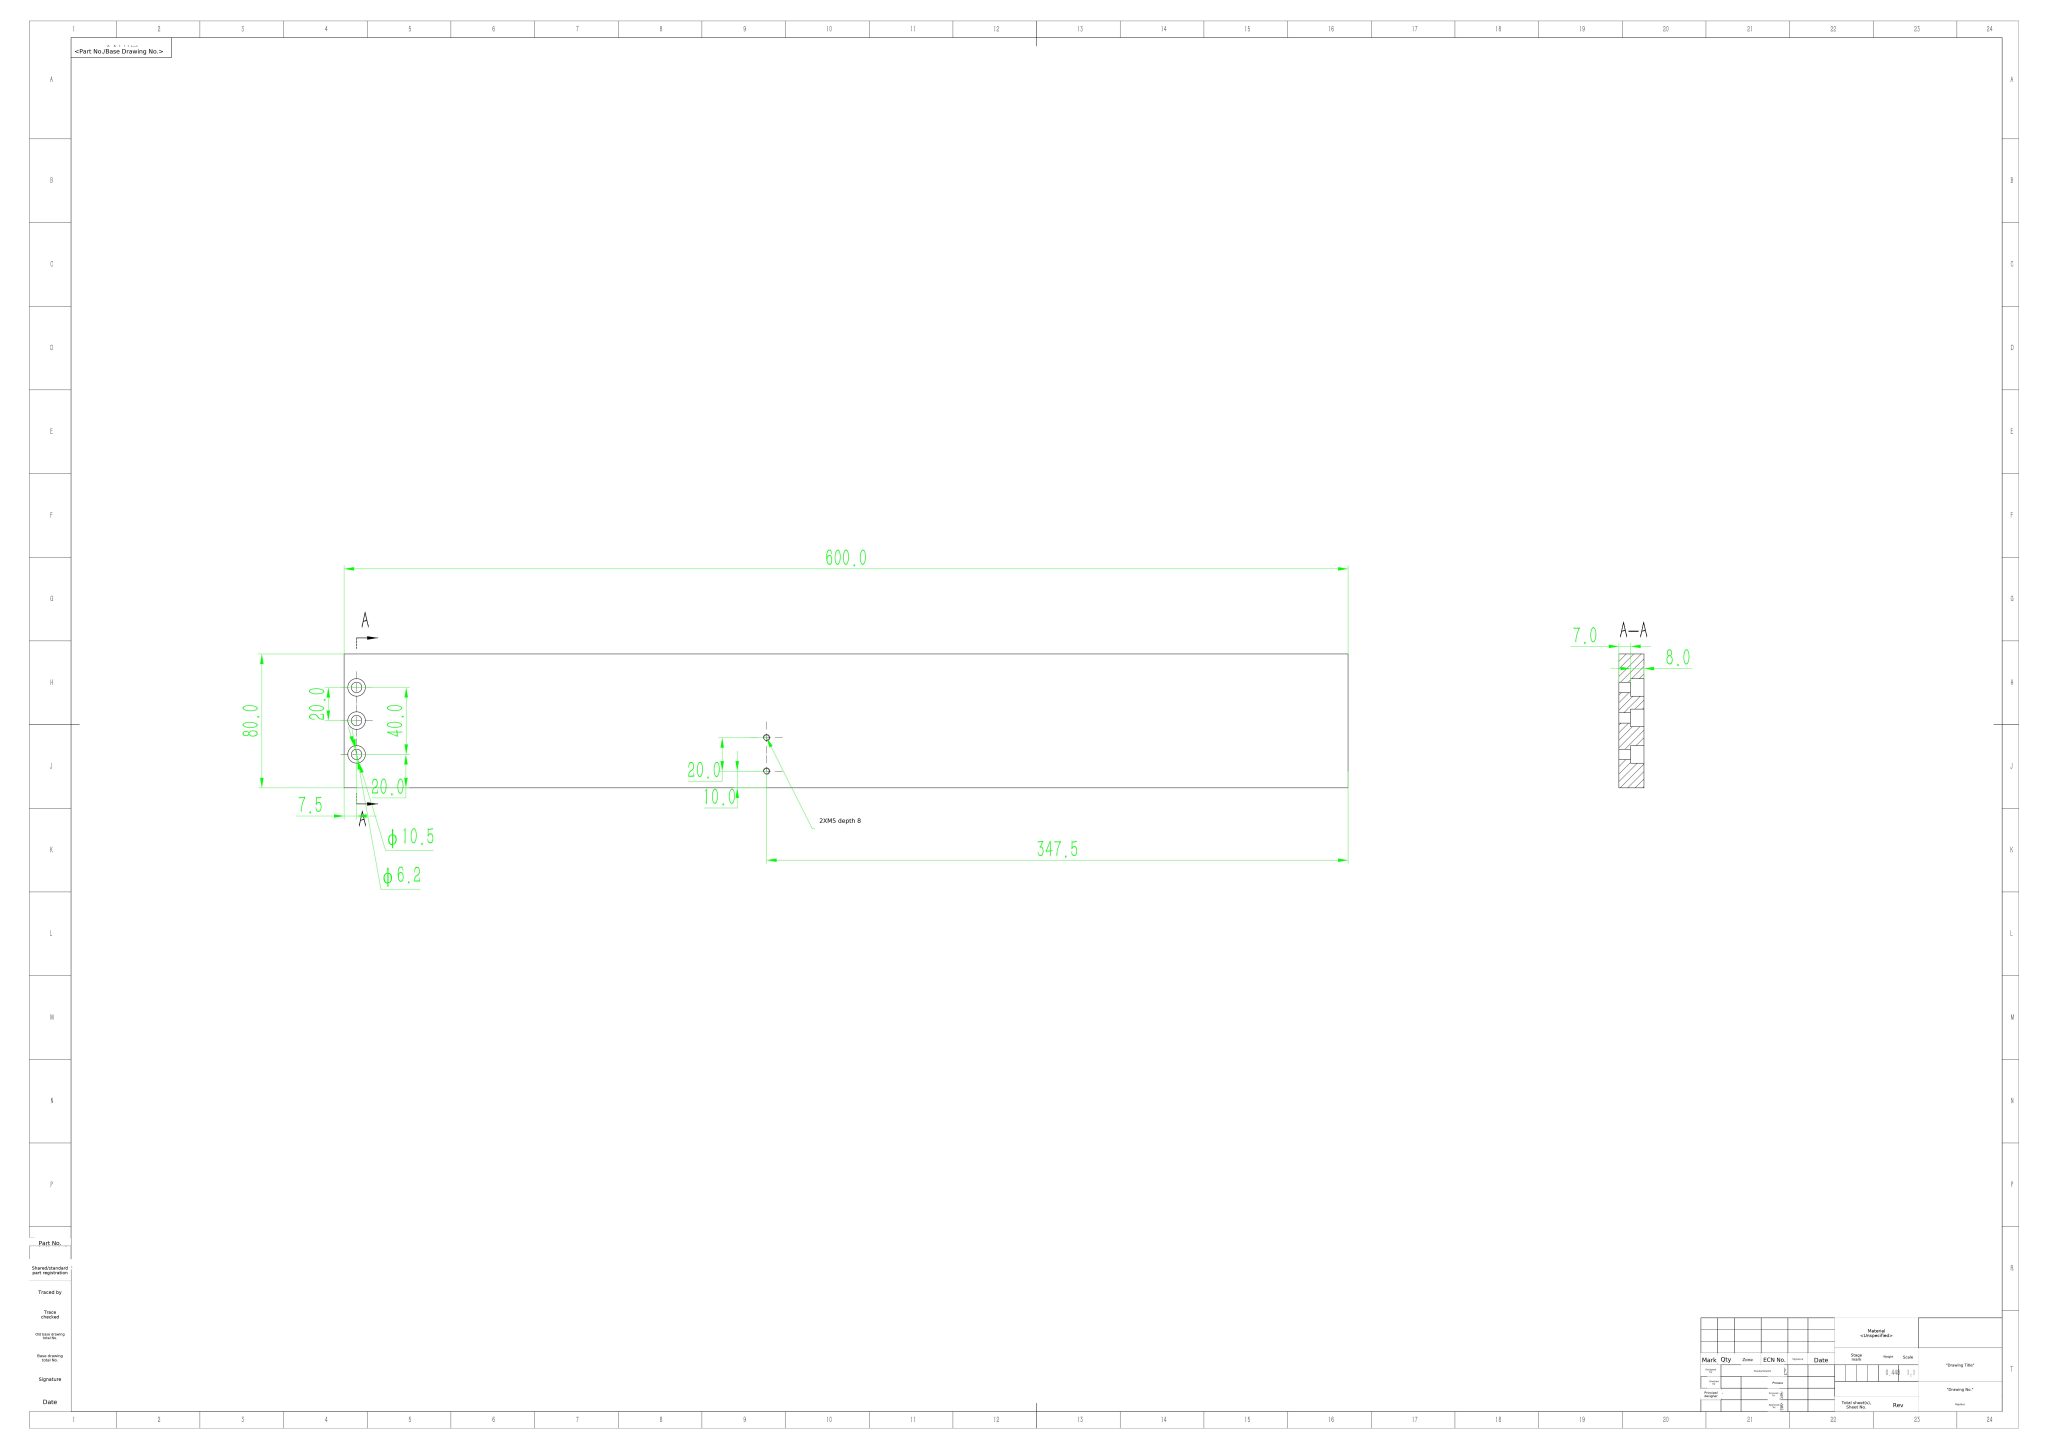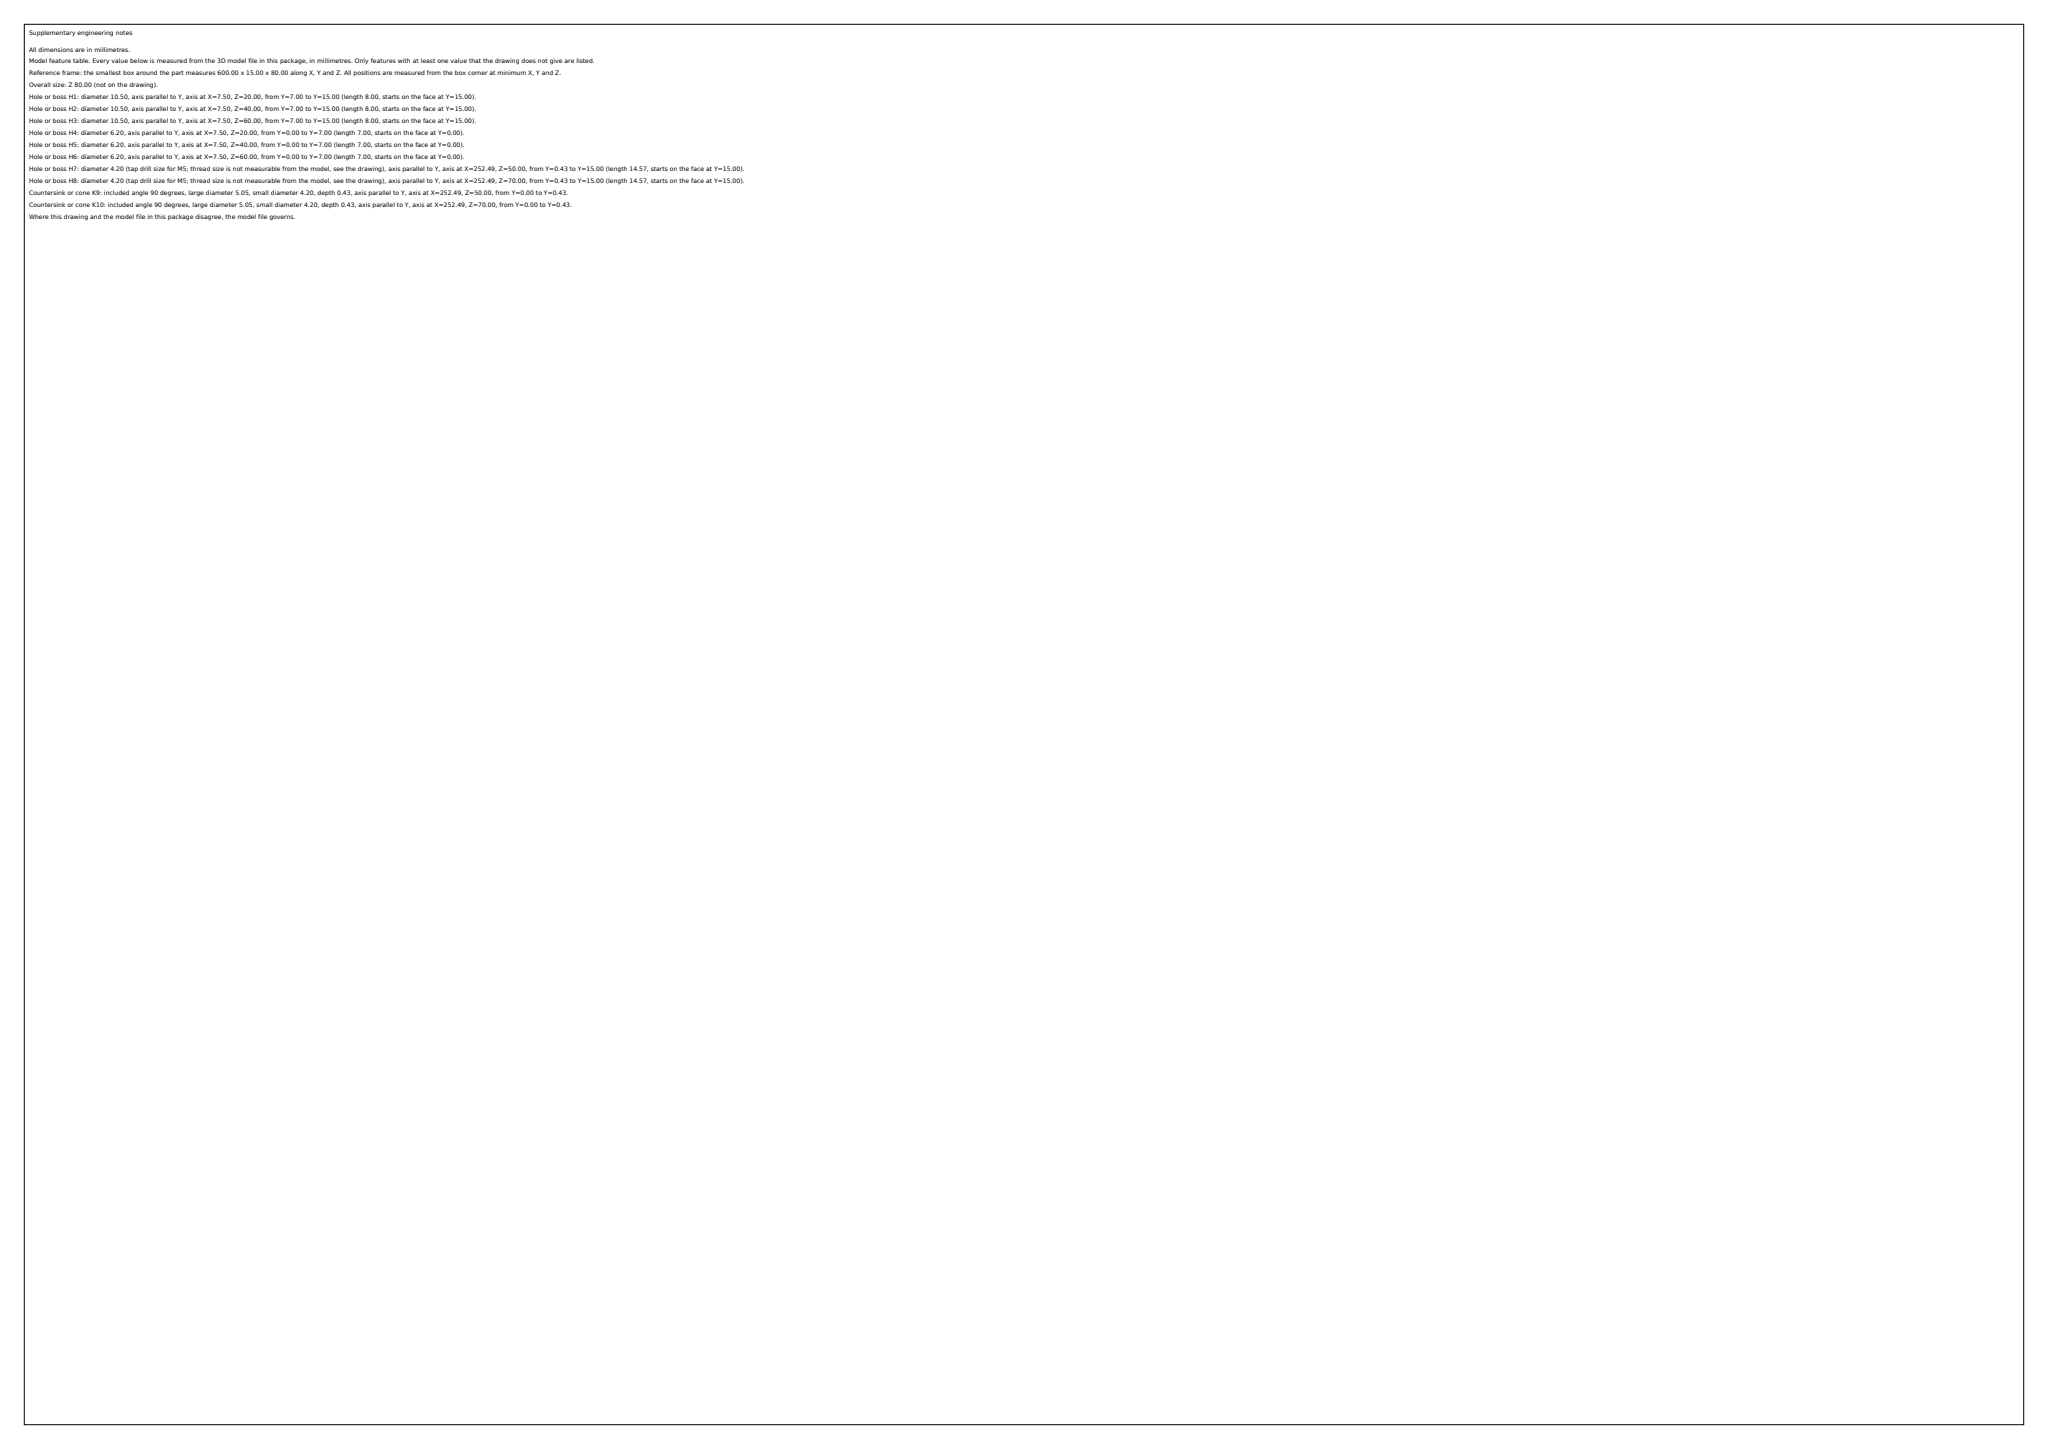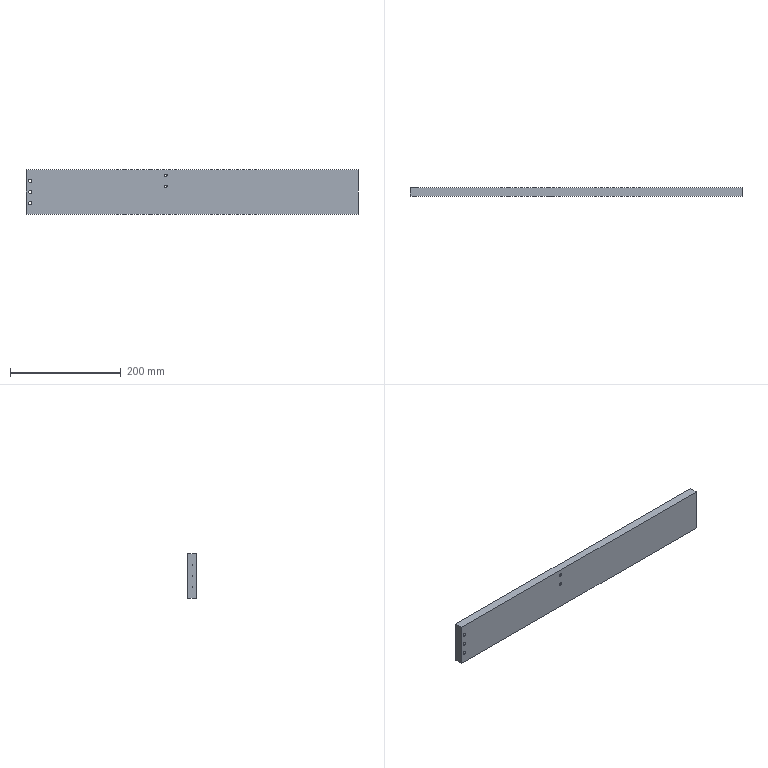Part | SolidWorks | mm | 1 solid | 29 faces | box 600 x 15 x 80 mm | volume 716870 mm3 | cylinder 16 | plane 9 | cone 4 | commonest cylinder face diameters 6.2 x6 10.5 x6 4.2 x4
build123d program:
from build123d import *

# Parameters (mm, degrees)
SKETCH1_W                   = 600
SKETCH1_H                   = 80
BOSS_EXTRUDE1_DEPTH         = 15
SKETCH2_R                   = 5.25
CUT_EXTRUDE1_DEPTH          = 8
SKETCH3_R                   = 3.1
CUT_EXTRUDE2_DEPTH          = 303.761
M5_TAPPED_HOLE1_D           = 4.2
M5_TAPPED_HOLE1_CSINK_D     = 5.05
M5_TAPPED_HOLE1_CSINK_ANGLE = 90


with BuildPart() as part:
    # Sketch1 → Boss-Extrude1 (new body)
    with BuildSketch(Plane(origin=(0, 0, 0), x_dir=(1, 0, 0), z_dir=(0, 1, 0))):
        Rectangle(SKETCH1_W, SKETCH1_H)
    extrude(amount=BOSS_EXTRUDE1_DEPTH)

    # Sketch2 → Cut-Extrude1 (cut)
    with BuildSketch(Plane(origin=(0, 15, 0), x_dir=(1, 0, 0), z_dir=(0, 1, 0))):
        with Locations(Location((-292.5, 20, 0), (0, 0, 270))):
            Circle(SKETCH2_R)
        with Locations(Location((-292.5, -20, 0), (0, 0, 270))):
            Circle(SKETCH2_R)
        with Locations(Location((-292.5, 0, 0), (0, 0, 270))):
            Circle(SKETCH2_R)
    extrude(amount=-CUT_EXTRUDE1_DEPTH, mode=Mode.SUBTRACT)

    # Sketch3 → Cut-Extrude2 (cut, through all)
    with BuildSketch(Plane(origin=(0, 7, 0), x_dir=(1, 0, 0), z_dir=(0, 1, 0))):
        with Locations(Location((-292.5, 20, 0), (0, 0, 270))):
            Circle(SKETCH3_R)
        with Locations(Location((-292.5, -20, 0), (0, 0, 270))):
            Circle(SKETCH3_R)
        with Locations(Location((-292.5, 0, 0), (0, 0, 270))):
            Circle(SKETCH3_R)
    extrude(amount=-CUT_EXTRUDE2_DEPTH, mode=Mode.SUBTRACT)

    # M5 Tapped Hole1 (through all)
    with Locations(Plane(origin=(0, 0, 0), x_dir=(-1, 0, 0), z_dir=(0, -1, 0))):
        with Locations((47.513, -30), (47.513, -10)):
            CounterSinkHole(M5_TAPPED_HOLE1_D / 2, M5_TAPPED_HOLE1_CSINK_D / 2, counter_sink_angle=M5_TAPPED_HOLE1_CSINK_ANGLE)


solid = part.part
STEP:
#1=CARTESIAN_POINT('',(-47.513,0.425,32.1));
#2=VERTEX_POINT('',#1);
#3=CARTESIAN_POINT('',(-47.513,0.425,27.9));
#4=VERTEX_POINT('',#3);
#5=CARTESIAN_POINT('',(-47.513,0.425,30.));
#6=DIRECTION('',(0.,-1.,0.));
#7=DIRECTION('',(0.,0.,-1.));
#8=AXIS2_PLACEMENT_3D('',#5,#6,#7);
#9=CIRCLE('',#8,2.1);
#10=EDGE_CURVE('',#2,#4,#9,.T.);
#11=ORIENTED_EDGE('',*,*,#10,.F.);
#12=CARTESIAN_POINT('',(-47.513,-0.,32.525));
#13=VERTEX_POINT('',#12);
#14=CARTESIAN_POINT('',(-47.513,-0.,32.525));
#15=DIRECTION('',(0.,-0.7071,0.7071));
#16=VECTOR('',#15,1000.);
#17=LINE('',#14,#16);
#18=EDGE_CURVE('',#2,#13,#17,.T.);
#19=ORIENTED_EDGE('',*,*,#18,.T.);
#20=CARTESIAN_POINT('',(-47.513,-0.,27.475));
#21=VERTEX_POINT('',#20);
#22=CARTESIAN_POINT('',(-47.513,-0.,30.));
#23=DIRECTION('',(0.,-1.,0.));
#24=DIRECTION('',(0.,0.,-1.));
#25=AXIS2_PLACEMENT_3D('',#22,#23,#24);
#26=CIRCLE('',#25,2.525);
#27=EDGE_CURVE('',#13,#21,#26,.T.);
#28=ORIENTED_EDGE('',*,*,#27,.T.);
#29=CARTESIAN_POINT('',(-47.513,-0.,27.475));
#30=DIRECTION('',(0.,-0.7071,-0.7071));
#31=VECTOR('',#30,1000.);
#32=LINE('',#29,#31);
#33=EDGE_CURVE('',#4,#21,#32,.T.);
#34=ORIENTED_EDGE('',*,*,#33,.F.);
#35=EDGE_LOOP('',(#11,#19,#28,#34));
#36=FACE_OUTER_BOUND('',#35,.T.);
#37=CARTESIAN_POINT('',(-47.513,-0.,30.));
#38=DIRECTION('',(0.,-1.,0.));
#39=DIRECTION('',(0.,0.,-1.));
#40=AXIS2_PLACEMENT_3D('',#37,#38,#39);
#41=CONICAL_SURFACE('',#40,2.525,0.7854);
#42=ADVANCED_FACE('',(#36),#41,.F.);
#43=CARTESIAN_POINT('',(-47.513,15.,32.1));
#44=VERTEX_POINT('',#43);
#45=CARTESIAN_POINT('',(-47.513,15.,27.9));
#46=VERTEX_POINT('',#45);
#47=CARTESIAN_POINT('',(-47.513,15.,30.));
#48=DIRECTION('',(0.,-1.,0.));
#49=DIRECTION('',(0.,0.,-1.));
#50=AXIS2_PLACEMENT_3D('',#47,#48,#49);
#51=CIRCLE('',#50,2.1);
#52=EDGE_CURVE('',#44,#46,#51,.T.);
#53=ORIENTED_EDGE('',*,*,#52,.F.);
#54=CARTESIAN_POINT('',(-47.513,0.,32.1));
#55=DIRECTION('',(0.,-1.,0.));
#56=VECTOR('',#55,1000.);
#57=LINE('',#54,#56);
#58=EDGE_CURVE('',#44,#2,#57,.T.);
#59=ORIENTED_EDGE('',*,*,#58,.T.);
#60=ORIENTED_EDGE('',*,*,#10,.T.);
#61=CARTESIAN_POINT('',(-47.513,0.,27.9));
#62=DIRECTION('',(0.,-1.,0.));
#63=VECTOR('',#62,1000.);
#64=LINE('',#61,#63);
#65=EDGE_CURVE('',#46,#4,#64,.T.);
#66=ORIENTED_EDGE('',*,*,#65,.F.);
#67=EDGE_LOOP('',(#53,#59,#60,#66));
#68=FACE_OUTER_BOUND('',#67,.T.);
#69=CARTESIAN_POINT('',(-47.513,0.,30.));
#70=DIRECTION('',(0.,-1.,0.));
#71=DIRECTION('',(0.,0.,-1.));
#72=AXIS2_PLACEMENT_3D('',#69,#70,#71);
#73=CYLINDRICAL_SURFACE('',#72,2.1);
#74=ADVANCED_FACE('',(#68),#73,.F.);
#75=CARTESIAN_POINT('',(-47.513,0.425,12.1));
#76=VERTEX_POINT('',#75);
#77=CARTESIAN_POINT('',(-47.513,0.425,7.9));
#78=VERTEX_POINT('',#77);
#79=CARTESIAN_POINT('',(-47.513,0.425,10.));
#80=DIRECTION('',(0.,-1.,0.));
#81=DIRECTION('',(0.,0.,-1.));
#82=AXIS2_PLACEMENT_3D('',#79,#80,#81);
#83=CIRCLE('',#82,2.1);
#84=EDGE_CURVE('',#76,#78,#83,.T.);
#85=ORIENTED_EDGE('',*,*,#84,.F.);
#86=CARTESIAN_POINT('',(-47.513,-0.,12.525));
#87=VERTEX_POINT('',#86);
#88=CARTESIAN_POINT('',(-47.513,-0.,12.525));
#89=DIRECTION('',(0.,-0.7071,0.7071));
#90=VECTOR('',#89,1000.);
#91=LINE('',#88,#90);
#92=EDGE_CURVE('',#76,#87,#91,.T.);
#93=ORIENTED_EDGE('',*,*,#92,.T.);
#94=CARTESIAN_POINT('',(-47.513,-0.,7.475));
#95=VERTEX_POINT('',#94);
#96=CARTESIAN_POINT('',(-47.513,-0.,10.));
#97=DIRECTION('',(0.,-1.,0.));
#98=DIRECTION('',(0.,0.,-1.));
#99=AXIS2_PLACEMENT_3D('',#96,#97,#98);
#100=CIRCLE('',#99,2.525);
#101=EDGE_CURVE('',#87,#95,#100,.T.);
#102=ORIENTED_EDGE('',*,*,#101,.T.);
#103=CARTESIAN_POINT('',(-47.513,-0.,7.475));
#104=DIRECTION('',(0.,-0.7071,-0.7071));
#105=VECTOR('',#104,1000.);
#106=LINE('',#103,#105);
#107=EDGE_CURVE('',#78,#95,#106,.T.);
#108=ORIENTED_EDGE('',*,*,#107,.F.);
#109=EDGE_LOOP('',(#85,#93,#102,#108));
#110=FACE_OUTER_BOUND('',#109,.T.);
#111=CARTESIAN_POINT('',(-47.513,-0.,10.));
#112=DIRECTION('',(0.,-1.,0.));
#113=DIRECTION('',(0.,0.,-1.));
#114=AXIS2_PLACEMENT_3D('',#111,#112,#113);
#115=CONICAL_SURFACE('',#114,2.525,0.7854);
#116=ADVANCED_FACE('',(#110),#115,.F.);
#117=CARTESIAN_POINT('',(-47.513,15.,12.1));
#118=VERTEX_POINT('',#117);
#119=CARTESIAN_POINT('',(-47.513,15.,7.9));
#120=VERTEX_POINT('',#119);
#121=CARTESIAN_POINT('',(-47.513,15.,10.));
#122=DIRECTION('',(0.,-1.,0.));
#123=DIRECTION('',(0.,0.,-1.));
#124=AXIS2_PLACEMENT_3D('',#121,#122,#123);
#125=CIRCLE('',#124,2.1);
#126=EDGE_CURVE('',#118,#120,#125,.T.);
#127=ORIENTED_EDGE('',*,*,#126,.F.);
#128=CARTESIAN_POINT('',(-47.513,0.,12.1));
#129=DIRECTION('',(0.,-1.,0.));
#130=VECTOR('',#129,1000.);
#131=LINE('',#128,#130);
#132=EDGE_CURVE('',#118,#76,#131,.T.);
#133=ORIENTED_EDGE('',*,*,#132,.T.);
#134=ORIENTED_EDGE('',*,*,#84,.T.);
#135=CARTESIAN_POINT('',(-47.513,0.,7.9));
#136=DIRECTION('',(0.,-1.,0.));
#137=VECTOR('',#136,1000.);
#138=LINE('',#135,#137);
#139=EDGE_CURVE('',#120,#78,#138,.T.);
#140=ORIENTED_EDGE('',*,*,#139,.F.);
#141=EDGE_LOOP('',(#127,#133,#134,#140));
#142=FACE_OUTER_BOUND('',#141,.T.);
#143=CARTESIAN_POINT('',(-47.513,0.,10.));
#144=DIRECTION('',(0.,-1.,0.));
#145=DIRECTION('',(0.,0.,-1.));
#146=AXIS2_PLACEMENT_3D('',#143,#144,#145);
#147=CYLINDRICAL_SURFACE('',#146,2.1);
#148=ADVANCED_FACE('',(#142),#147,.F.);
#149=CARTESIAN_POINT('',(-292.5,0.,-23.1));
#150=VERTEX_POINT('',#149);
#151=CARTESIAN_POINT('',(-292.5,0.,-16.9));
#152=VERTEX_POINT('',#151);
#153=CARTESIAN_POINT('',(-292.5,0.,-20.));
#154=DIRECTION('',(0.,1.,0.));
#155=DIRECTION('',(0.,0.,1.));
#156=AXIS2_PLACEMENT_3D('',#153,#154,#155);
#157=CIRCLE('',#156,3.1);
#158=EDGE_CURVE('',#150,#152,#157,.T.);
#159=ORIENTED_EDGE('',*,*,#158,.F.);
#160=CARTESIAN_POINT('',(-292.5,7.,-23.1));
#161=VERTEX_POINT('',#160);
#162=CARTESIAN_POINT('',(-292.5,0.,-23.1));
#163=DIRECTION('',(0.,1.,0.));
#164=VECTOR('',#163,1000.);
#165=LINE('',#162,#164);
#166=EDGE_CURVE('',#150,#161,#165,.T.);
#167=ORIENTED_EDGE('',*,*,#166,.T.);
#168=CARTESIAN_POINT('',(-292.5,7.,-16.9));
#169=VERTEX_POINT('',#168);
#170=CARTESIAN_POINT('',(-292.5,7.,-20.));
#171=DIRECTION('',(0.,1.,0.));
#172=DIRECTION('',(0.,0.,1.));
#173=AXIS2_PLACEMENT_3D('',#170,#171,#172);
#174=CIRCLE('',#173,3.1);
#175=EDGE_CURVE('',#161,#169,#174,.T.);
#176=ORIENTED_EDGE('',*,*,#175,.T.);
#177=CARTESIAN_POINT('',(-292.5,0.,-16.9));
#178=DIRECTION('',(0.,1.,0.));
#179=VECTOR('',#178,1000.);
#180=LINE('',#177,#179);
#181=EDGE_CURVE('',#152,#169,#180,.T.);
#182=ORIENTED_EDGE('',*,*,#181,.F.);
#183=EDGE_LOOP('',(#159,#167,#176,#182));
#184=FACE_OUTER_BOUND('',#183,.T.);
#185=CARTESIAN_POINT('',(-292.5,0.,-20.));
#186=DIRECTION('',(0.,1.,0.));
#187=DIRECTION('',(0.,0.,1.));
#188=AXIS2_PLACEMENT_3D('',#185,#186,#187);
#189=CYLINDRICAL_SURFACE('',#188,3.1);
#190=ADVANCED_FACE('',(#184),#189,.F.);
#191=CARTESIAN_POINT('',(-292.5,0.,16.9));
#192=VERTEX_POINT('',#191);
#193=CARTESIAN_POINT('',(-292.5,0.,23.1));
#194=VERTEX_POINT('',#193);
#195=CARTESIAN_POINT('',(-292.5,0.,20.));
#196=DIRECTION('',(0.,1.,0.));
#197=DIRECTION('',(0.,0.,1.));
#198=AXIS2_PLACEMENT_3D('',#195,#196,#197);
#199=CIRCLE('',#198,3.1);
#200=EDGE_CURVE('',#192,#194,#199,.T.);
#201=ORIENTED_EDGE('',*,*,#200,.F.);
#202=CARTESIAN_POINT('',(-292.5,7.,16.9));
#203=VERTEX_POINT('',#202);
#204=CARTESIAN_POINT('',(-292.5,0.,16.9));
#205=DIRECTION('',(0.,1.,0.));
#206=VECTOR('',#205,1000.);
#207=LINE('',#204,#206);
#208=EDGE_CURVE('',#192,#203,#207,.T.);
#209=ORIENTED_EDGE('',*,*,#208,.T.);
#210=CARTESIAN_POINT('',(-292.5,7.,23.1));
#211=VERTEX_POINT('',#210);
#212=CARTESIAN_POINT('',(-292.5,7.,20.));
#213=DIRECTION('',(0.,1.,0.));
#214=DIRECTION('',(0.,0.,1.));
#215=AXIS2_PLACEMENT_3D('',#212,#213,#214);
#216=CIRCLE('',#215,3.1);
#217=EDGE_CURVE('',#203,#211,#216,.T.);
#218=ORIENTED_EDGE('',*,*,#217,.T.);
#219=CARTESIAN_POINT('',(-292.5,0.,23.1));
#220=DIRECTION('',(0.,1.,0.));
#221=VECTOR('',#220,1000.);
#222=LINE('',#219,#221);
#223=EDGE_CURVE('',#194,#211,#222,.T.);
#224=ORIENTED_EDGE('',*,*,#223,.F.);
#225=EDGE_LOOP('',(#201,#209,#218,#224));
#226=FACE_OUTER_BOUND('',#225,.T.);
#227=CARTESIAN_POINT('',(-292.5,0.,20.));
#228=DIRECTION('',(0.,1.,0.));
#229=DIRECTION('',(0.,0.,1.));
#230=AXIS2_PLACEMENT_3D('',#227,#228,#229);
#231=CYLINDRICAL_SURFACE('',#230,3.1);
#232=ADVANCED_FACE('',(#226),#231,.F.);
#233=CARTESIAN_POINT('',(-292.5,0.,-3.1));
#234=VERTEX_POINT('',#233);
#235=CARTESIAN_POINT('',(-292.5,0.,3.1));
#236=VERTEX_POINT('',#235);
#237=CARTESIAN_POINT('',(-292.5,0.,0.));
#238=DIRECTION('',(0.,1.,0.));
#239=DIRECTION('',(0.,0.,1.));
#240=AXIS2_PLACEMENT_3D('',#237,#238,#239);
#241=CIRCLE('',#240,3.1);
#242=EDGE_CURVE('',#234,#236,#241,.T.);
#243=ORIENTED_EDGE('',*,*,#242,.F.);
#244=CARTESIAN_POINT('',(-292.5,7.,-3.1));
#245=VERTEX_POINT('',#244);
#246=CARTESIAN_POINT('',(-292.5,0.,-3.1));
#247=DIRECTION('',(0.,1.,0.));
#248=VECTOR('',#247,1000.);
#249=LINE('',#246,#248);
#250=EDGE_CURVE('',#234,#245,#249,.T.);
#251=ORIENTED_EDGE('',*,*,#250,.T.);
#252=CARTESIAN_POINT('',(-292.5,7.,3.1));
#253=VERTEX_POINT('',#252);
#254=CARTESIAN_POINT('',(-292.5,7.,0.));
#255=DIRECTION('',(0.,1.,0.));
#256=DIRECTION('',(0.,0.,1.));
#257=AXIS2_PLACEMENT_3D('',#254,#255,#256);
#258=CIRCLE('',#257,3.1);
#259=EDGE_CURVE('',#245,#253,#258,.T.);
#260=ORIENTED_EDGE('',*,*,#259,.T.);
#261=CARTESIAN_POINT('',(-292.5,0.,3.1));
#262=DIRECTION('',(0.,1.,0.));
#263=VECTOR('',#262,1000.);
#264=LINE('',#261,#263);
#265=EDGE_CURVE('',#236,#253,#264,.T.);
#266=ORIENTED_EDGE('',*,*,#265,.F.);
#267=EDGE_LOOP('',(#243,#251,#260,#266));
#268=FACE_OUTER_BOUND('',#267,.T.);
#269=CARTESIAN_POINT('',(-292.5,0.,0.));
#270=DIRECTION('',(0.,1.,0.));
#271=DIRECTION('',(0.,0.,1.));
#272=AXIS2_PLACEMENT_3D('',#269,#270,#271);
#273=CYLINDRICAL_SURFACE('',#272,3.1);
#274=ADVANCED_FACE('',(#268),#273,.F.);
#275=CARTESIAN_POINT('',(-292.5,7.,-25.25));
#276=VERTEX_POINT('',#275);
#277=CARTESIAN_POINT('',(-292.5,7.,-14.75));
#278=VERTEX_POINT('',#277);
#279=CARTESIAN_POINT('',(-292.5,7.,-20.));
#280=DIRECTION('',(0.,1.,0.));
#281=DIRECTION('',(0.,0.,1.));
#282=AXIS2_PLACEMENT_3D('',#279,#280,#281);
#283=CIRCLE('',#282,5.25);
#284=EDGE_CURVE('',#276,#278,#283,.T.);
#285=ORIENTED_EDGE('',*,*,#284,.F.);
#286=CARTESIAN_POINT('',(-292.5,15.,-25.25));
#287=VERTEX_POINT('',#286);
#288=CARTESIAN_POINT('',(-292.5,7.,-25.25));
#289=DIRECTION('',(0.,1.,0.));
#290=VECTOR('',#289,1000.);
#291=LINE('',#288,#290);
#292=EDGE_CURVE('',#276,#287,#291,.T.);
#293=ORIENTED_EDGE('',*,*,#292,.T.);
#294=CARTESIAN_POINT('',(-292.5,15.,-14.75));
#295=VERTEX_POINT('',#294);
#296=CARTESIAN_POINT('',(-292.5,15.,-20.));
#297=DIRECTION('',(0.,1.,0.));
#298=DIRECTION('',(0.,0.,1.));
#299=AXIS2_PLACEMENT_3D('',#296,#297,#298);
#300=CIRCLE('',#299,5.25);
#301=EDGE_CURVE('',#287,#295,#300,.T.);
#302=ORIENTED_EDGE('',*,*,#301,.T.);
#303=CARTESIAN_POINT('',(-292.5,7.,-14.75));
#304=DIRECTION('',(0.,1.,0.));
#305=VECTOR('',#304,1000.);
#306=LINE('',#303,#305);
#307=EDGE_CURVE('',#278,#295,#306,.T.);
#308=ORIENTED_EDGE('',*,*,#307,.F.);
#309=EDGE_LOOP('',(#285,#293,#302,#308));
#310=FACE_OUTER_BOUND('',#309,.T.);
#311=CARTESIAN_POINT('',(-292.5,7.,-20.));
#312=DIRECTION('',(0.,1.,0.));
#313=DIRECTION('',(0.,0.,1.));
#314=AXIS2_PLACEMENT_3D('',#311,#312,#313);
#315=CYLINDRICAL_SURFACE('',#314,5.25);
#316=ADVANCED_FACE('',(#310),#315,.F.);
#317=CARTESIAN_POINT('',(-292.5,7.,14.75));
#318=VERTEX_POINT('',#317);
#319=CARTESIAN_POINT('',(-292.5,7.,25.25));
#320=VERTEX_POINT('',#319);
#321=CARTESIAN_POINT('',(-292.5,7.,20.));
#322=DIRECTION('',(0.,1.,0.));
#323=DIRECTION('',(0.,0.,1.));
#324=AXIS2_PLACEMENT_3D('',#321,#322,#323);
#325=CIRCLE('',#324,5.25);
#326=EDGE_CURVE('',#318,#320,#325,.T.);
#327=ORIENTED_EDGE('',*,*,#326,.F.);
#328=CARTESIAN_POINT('',(-292.5,15.,14.75));
#329=VERTEX_POINT('',#328);
#330=CARTESIAN_POINT('',(-292.5,7.,14.75));
#331=DIRECTION('',(0.,1.,0.));
#332=VECTOR('',#331,1000.);
#333=LINE('',#330,#332);
#334=EDGE_CURVE('',#318,#329,#333,.T.);
#335=ORIENTED_EDGE('',*,*,#334,.T.);
#336=CARTESIAN_POINT('',(-292.5,15.,25.25));
#337=VERTEX_POINT('',#336);
#338=CARTESIAN_POINT('',(-292.5,15.,20.));
#339=DIRECTION('',(0.,1.,0.));
#340=DIRECTION('',(0.,0.,1.));
#341=AXIS2_PLACEMENT_3D('',#338,#339,#340);
#342=CIRCLE('',#341,5.25);
#343=EDGE_CURVE('',#329,#337,#342,.T.);
#344=ORIENTED_EDGE('',*,*,#343,.T.);
#345=CARTESIAN_POINT('',(-292.5,7.,25.25));
#346=DIRECTION('',(0.,1.,0.));
#347=VECTOR('',#346,1000.);
#348=LINE('',#345,#347);
#349=EDGE_CURVE('',#320,#337,#348,.T.);
#350=ORIENTED_EDGE('',*,*,#349,.F.);
#351=EDGE_LOOP('',(#327,#335,#344,#350));
#352=FACE_OUTER_BOUND('',#351,.T.);
#353=CARTESIAN_POINT('',(-292.5,7.,20.));
#354=DIRECTION('',(0.,1.,0.));
#355=DIRECTION('',(0.,0.,1.));
#356=AXIS2_PLACEMENT_3D('',#353,#354,#355);
#357=CYLINDRICAL_SURFACE('',#356,5.25);
#358=ADVANCED_FACE('',(#352),#357,.F.);
#359=CARTESIAN_POINT('',(-292.5,7.,-5.25));
#360=VERTEX_POINT('',#359);
#361=CARTESIAN_POINT('',(-292.5,7.,5.25));
#362=VERTEX_POINT('',#361);
#363=CARTESIAN_POINT('',(-292.5,7.,0.));
#364=DIRECTION('',(0.,1.,0.));
#365=DIRECTION('',(0.,0.,1.));
#366=AXIS2_PLACEMENT_3D('',#363,#364,#365);
#367=CIRCLE('',#366,5.25);
#368=EDGE_CURVE('',#360,#362,#367,.T.);
#369=ORIENTED_EDGE('',*,*,#368,.F.);
#370=CARTESIAN_POINT('',(-292.5,15.,-5.25));
#371=VERTEX_POINT('',#370);
#372=CARTESIAN_POINT('',(-292.5,7.,-5.25));
#373=DIRECTION('',(0.,1.,0.));
#374=VECTOR('',#373,1000.);
#375=LINE('',#372,#374);
#376=EDGE_CURVE('',#360,#371,#375,.T.);
#377=ORIENTED_EDGE('',*,*,#376,.T.);
#378=CARTESIAN_POINT('',(-292.5,15.,5.25));
#379=VERTEX_POINT('',#378);
#380=CARTESIAN_POINT('',(-292.5,15.,0.));
#381=DIRECTION('',(0.,1.,0.));
#382=DIRECTION('',(0.,0.,1.));
#383=AXIS2_PLACEMENT_3D('',#380,#381,#382);
#384=CIRCLE('',#383,5.25);
#385=EDGE_CURVE('',#371,#379,#384,.T.);
#386=ORIENTED_EDGE('',*,*,#385,.T.);
#387=CARTESIAN_POINT('',(-292.5,7.,5.25));
#388=DIRECTION('',(0.,1.,0.));
#389=VECTOR('',#388,1000.);
#390=LINE('',#387,#389);
#391=EDGE_CURVE('',#362,#379,#390,.T.);
#392=ORIENTED_EDGE('',*,*,#391,.F.);
#393=EDGE_LOOP('',(#369,#377,#386,#392));
#394=FACE_OUTER_BOUND('',#393,.T.);
#395=CARTESIAN_POINT('',(-292.5,7.,0.));
#396=DIRECTION('',(0.,1.,0.));
#397=DIRECTION('',(0.,0.,1.));
#398=AXIS2_PLACEMENT_3D('',#395,#396,#397);
#399=CYLINDRICAL_SURFACE('',#398,5.25);
#400=ADVANCED_FACE('',(#394),#399,.F.);
#401=CARTESIAN_POINT('',(300.,0.,40.));
#402=VERTEX_POINT('',#401);
#403=CARTESIAN_POINT('',(300.,0.,-40.));
#404=VERTEX_POINT('',#403);
#405=CARTESIAN_POINT('',(300.,0.,40.));
#406=DIRECTION('',(0.,0.,-1.));
#407=VECTOR('',#406,1000.);
#408=LINE('',#405,#407);
#409=EDGE_CURVE('',#402,#404,#408,.T.);
#410=ORIENTED_EDGE('',*,*,#409,.T.);
#411=CARTESIAN_POINT('',(300.,15.,-40.));
#412=VERTEX_POINT('',#411);
#413=CARTESIAN_POINT('',(300.,15.,-40.));
#414=DIRECTION('',(0.,-1.,0.));
#415=VECTOR('',#414,1000.);
#416=LINE('',#413,#415);
#417=EDGE_CURVE('',#412,#404,#416,.T.);
#418=ORIENTED_EDGE('',*,*,#417,.F.);
#419=CARTESIAN_POINT('',(300.,15.,40.));
#420=VERTEX_POINT('',#419);
#421=CARTESIAN_POINT('',(300.,15.,40.));
#422=DIRECTION('',(0.,0.,-1.));
#423=VECTOR('',#422,1000.);
#424=LINE('',#421,#423);
#425=EDGE_CURVE('',#420,#412,#424,.T.);
#426=ORIENTED_EDGE('',*,*,#425,.F.);
#427=CARTESIAN_POINT('',(300.,15.,40.));
#428=DIRECTION('',(0.,-1.,0.));
#429=VECTOR('',#428,1000.);
#430=LINE('',#427,#429);
#431=EDGE_CURVE('',#420,#402,#430,.T.);
#432=ORIENTED_EDGE('',*,*,#431,.T.);
#433=EDGE_LOOP('',(#410,#418,#426,#432));
#434=FACE_OUTER_BOUND('',#433,.T.);
#435=CARTESIAN_POINT('',(300.,15.,40.));
#436=DIRECTION('',(-1.,0.,0.));
#437=DIRECTION('',(0.,0.,1.));
#438=AXIS2_PLACEMENT_3D('',#435,#436,#437);
#439=PLANE('',#438);
#440=ADVANCED_FACE('',(#434),#439,.F.);
#441=CARTESIAN_POINT('',(-300.,0.,-40.));
#442=VERTEX_POINT('',#441);
#443=CARTESIAN_POINT('',(-300.,0.,-40.));
#444=DIRECTION('',(-1.,0.,0.));
#445=VECTOR('',#444,1000.);
#446=LINE('',#443,#445);
#447=EDGE_CURVE('',#404,#442,#446,.T.);
#448=ORIENTED_EDGE('',*,*,#447,.T.);
#449=CARTESIAN_POINT('',(-300.,15.,-40.));
#450=VERTEX_POINT('',#449);
#451=CARTESIAN_POINT('',(-300.,15.,-40.));
#452=DIRECTION('',(0.,-1.,0.));
#453=VECTOR('',#452,1000.);
#454=LINE('',#451,#453);
#455=EDGE_CURVE('',#450,#442,#454,.T.);
#456=ORIENTED_EDGE('',*,*,#455,.F.);
#457=CARTESIAN_POINT('',(-300.,15.,-40.));
#458=DIRECTION('',(-1.,0.,0.));
#459=VECTOR('',#458,1000.);
#460=LINE('',#457,#459);
#461=EDGE_CURVE('',#412,#450,#460,.T.);
#462=ORIENTED_EDGE('',*,*,#461,.F.);
#463=ORIENTED_EDGE('',*,*,#417,.T.);
#464=EDGE_LOOP('',(#448,#456,#462,#463));
#465=FACE_OUTER_BOUND('',#464,.T.);
#466=CARTESIAN_POINT('',(-300.,15.,-40.));
#467=DIRECTION('',(0.,0.,1.));
#468=DIRECTION('',(1.,0.,0.));
#469=AXIS2_PLACEMENT_3D('',#466,#467,#468);
#470=PLANE('',#469);
#471=ADVANCED_FACE('',(#465),#470,.F.);
#472=CARTESIAN_POINT('',(-300.,0.,40.));
#473=VERTEX_POINT('',#472);
#474=CARTESIAN_POINT('',(-300.,0.,40.));
#475=DIRECTION('',(0.,0.,1.));
#476=VECTOR('',#475,1000.);
#477=LINE('',#474,#476);
#478=EDGE_CURVE('',#442,#473,#477,.T.);
#479=ORIENTED_EDGE('',*,*,#478,.T.);
#480=CARTESIAN_POINT('',(-300.,15.,40.));
#481=VERTEX_POINT('',#480);
#482=CARTESIAN_POINT('',(-300.,15.,40.));
#483=DIRECTION('',(0.,-1.,0.));
#484=VECTOR('',#483,1000.);
#485=LINE('',#482,#484);
#486=EDGE_CURVE('',#481,#473,#485,.T.);
#487=ORIENTED_EDGE('',*,*,#486,.F.);
#488=CARTESIAN_POINT('',(-300.,15.,40.));
#489=DIRECTION('',(0.,0.,1.));
#490=VECTOR('',#489,1000.);
#491=LINE('',#488,#490);
#492=EDGE_CURVE('',#450,#481,#491,.T.);
#493=ORIENTED_EDGE('',*,*,#492,.F.);
#494=ORIENTED_EDGE('',*,*,#455,.T.);
#495=EDGE_LOOP('',(#479,#487,#493,#494));
#496=FACE_OUTER_BOUND('',#495,.T.);
#497=CARTESIAN_POINT('',(-300.,15.,40.));
#498=DIRECTION('',(1.,0.,0.));
#499=DIRECTION('',(0.,0.,-1.));
#500=AXIS2_PLACEMENT_3D('',#497,#498,#499);
#501=PLANE('',#500);
#502=ADVANCED_FACE('',(#496),#501,.F.);
#503=CARTESIAN_POINT('',(-300.,0.,40.));
#504=DIRECTION('',(1.,0.,0.));
#505=VECTOR('',#504,1000.);
#506=LINE('',#503,#505);
#507=EDGE_CURVE('',#473,#402,#506,.T.);
#508=ORIENTED_EDGE('',*,*,#507,.T.);
#509=ORIENTED_EDGE('',*,*,#431,.F.);
#510=CARTESIAN_POINT('',(-300.,15.,40.));
#511=DIRECTION('',(1.,0.,0.));
#512=VECTOR('',#511,1000.);
#513=LINE('',#510,#512);
#514=EDGE_CURVE('',#481,#420,#513,.T.);
#515=ORIENTED_EDGE('',*,*,#514,.F.);
#516=ORIENTED_EDGE('',*,*,#486,.T.);
#517=EDGE_LOOP('',(#508,#509,#515,#516));
#518=FACE_OUTER_BOUND('',#517,.T.);
#519=CARTESIAN_POINT('',(-300.,15.,40.));
#520=DIRECTION('',(0.,0.,-1.));
#521=DIRECTION('',(-1.,0.,0.));
#522=AXIS2_PLACEMENT_3D('',#519,#520,#521);
#523=PLANE('',#522);
#524=ADVANCED_FACE('',(#518),#523,.F.);
#525=CARTESIAN_POINT('',(-47.513,15.,30.));
#526=DIRECTION('',(0.,-1.,0.));
#527=DIRECTION('',(0.,0.,-1.));
#528=AXIS2_PLACEMENT_3D('',#525,#526,#527);
#529=CIRCLE('',#528,2.1);
#530=EDGE_CURVE('',#46,#44,#529,.T.);
#531=ORIENTED_EDGE('',*,*,#530,.T.);
#532=ORIENTED_EDGE('',*,*,#52,.T.);
#533=EDGE_LOOP('',(#531,#532));
#534=FACE_BOUND('',#533,.T.);
#535=CARTESIAN_POINT('',(-47.513,15.,10.));
#536=DIRECTION('',(0.,-1.,0.));
#537=DIRECTION('',(0.,0.,-1.));
#538=AXIS2_PLACEMENT_3D('',#535,#536,#537);
#539=CIRCLE('',#538,2.1);
#540=EDGE_CURVE('',#120,#118,#539,.T.);
#541=ORIENTED_EDGE('',*,*,#540,.T.);
#542=ORIENTED_EDGE('',*,*,#126,.T.);
#543=EDGE_LOOP('',(#541,#542));
#544=FACE_BOUND('',#543,.T.);
#545=CARTESIAN_POINT('',(-292.5,15.,-20.));
#546=DIRECTION('',(0.,1.,0.));
#547=DIRECTION('',(0.,0.,1.));
#548=AXIS2_PLACEMENT_3D('',#545,#546,#547);
#549=CIRCLE('',#548,5.25);
#550=EDGE_CURVE('',#295,#287,#549,.T.);
#551=ORIENTED_EDGE('',*,*,#550,.F.);
#552=ORIENTED_EDGE('',*,*,#301,.F.);
#553=EDGE_LOOP('',(#551,#552));
#554=FACE_BOUND('',#553,.T.);
#555=CARTESIAN_POINT('',(-292.5,15.,20.));
#556=DIRECTION('',(0.,1.,0.));
#557=DIRECTION('',(0.,0.,1.));
#558=AXIS2_PLACEMENT_3D('',#555,#556,#557);
#559=CIRCLE('',#558,5.25);
#560=EDGE_CURVE('',#337,#329,#559,.T.);
#561=ORIENTED_EDGE('',*,*,#560,.F.);
#562=ORIENTED_EDGE('',*,*,#343,.F.);
#563=EDGE_LOOP('',(#561,#562));
#564=FACE_BOUND('',#563,.T.);
#565=CARTESIAN_POINT('',(-292.5,15.,0.));
#566=DIRECTION('',(0.,1.,0.));
#567=DIRECTION('',(0.,0.,1.));
#568=AXIS2_PLACEMENT_3D('',#565,#566,#567);
#569=CIRCLE('',#568,5.25);
#570=EDGE_CURVE('',#379,#371,#569,.T.);
#571=ORIENTED_EDGE('',*,*,#570,.F.);
#572=ORIENTED_EDGE('',*,*,#385,.F.);
#573=EDGE_LOOP('',(#571,#572));
#574=FACE_BOUND('',#573,.T.);
#575=ORIENTED_EDGE('',*,*,#425,.T.);
#576=ORIENTED_EDGE('',*,*,#461,.T.);
#577=ORIENTED_EDGE('',*,*,#492,.T.);
#578=ORIENTED_EDGE('',*,*,#514,.T.);
#579=EDGE_LOOP('',(#575,#576,#577,#578));
#580=FACE_OUTER_BOUND('',#579,.T.);
#581=CARTESIAN_POINT('',(0.,15.,0.));
#582=DIRECTION('',(0.,-1.,0.));
#583=DIRECTION('',(0.,0.,-1.));
#584=AXIS2_PLACEMENT_3D('',#581,#582,#583);
#585=PLANE('',#584);
#586=ADVANCED_FACE('',(#534,#544,#554,#564,#574,#580),#585,.F.);
#587=CARTESIAN_POINT('',(-47.513,-0.,30.));
#588=DIRECTION('',(0.,-1.,0.));
#589=DIRECTION('',(0.,0.,-1.));
#590=AXIS2_PLACEMENT_3D('',#587,#588,#589);
#591=CIRCLE('',#590,2.525);
#592=EDGE_CURVE('',#21,#13,#591,.T.);
#593=ORIENTED_EDGE('',*,*,#592,.F.);
#594=ORIENTED_EDGE('',*,*,#27,.F.);
#595=EDGE_LOOP('',(#593,#594));
#596=FACE_BOUND('',#595,.T.);
#597=CARTESIAN_POINT('',(-47.513,-0.,10.));
#598=DIRECTION('',(0.,-1.,0.));
#599=DIRECTION('',(0.,0.,-1.));
#600=AXIS2_PLACEMENT_3D('',#597,#598,#599);
#601=CIRCLE('',#600,2.525);
#602=EDGE_CURVE('',#95,#87,#601,.T.);
#603=ORIENTED_EDGE('',*,*,#602,.F.);
#604=ORIENTED_EDGE('',*,*,#101,.F.);
#605=EDGE_LOOP('',(#603,#604));
#606=FACE_BOUND('',#605,.T.);
#607=CARTESIAN_POINT('',(-292.5,0.,-20.));
#608=DIRECTION('',(0.,1.,0.));
#609=DIRECTION('',(0.,0.,1.));
#610=AXIS2_PLACEMENT_3D('',#607,#608,#609);
#611=CIRCLE('',#610,3.1);
#612=EDGE_CURVE('',#152,#150,#611,.T.);
#613=ORIENTED_EDGE('',*,*,#612,.T.);
#614=ORIENTED_EDGE('',*,*,#158,.T.);
#615=EDGE_LOOP('',(#613,#614));
#616=FACE_BOUND('',#615,.T.);
#617=CARTESIAN_POINT('',(-292.5,0.,20.));
#618=DIRECTION('',(0.,1.,0.));
#619=DIRECTION('',(0.,0.,1.));
#620=AXIS2_PLACEMENT_3D('',#617,#618,#619);
#621=CIRCLE('',#620,3.1);
#622=EDGE_CURVE('',#194,#192,#621,.T.);
#623=ORIENTED_EDGE('',*,*,#622,.T.);
#624=ORIENTED_EDGE('',*,*,#200,.T.);
#625=EDGE_LOOP('',(#623,#624));
#626=FACE_BOUND('',#625,.T.);
#627=CARTESIAN_POINT('',(-292.5,0.,0.));
#628=DIRECTION('',(0.,1.,0.));
#629=DIRECTION('',(0.,0.,1.));
#630=AXIS2_PLACEMENT_3D('',#627,#628,#629);
#631=CIRCLE('',#630,3.1);
#632=EDGE_CURVE('',#236,#234,#631,.T.);
#633=ORIENTED_EDGE('',*,*,#632,.T.);
#634=ORIENTED_EDGE('',*,*,#242,.T.);
#635=EDGE_LOOP('',(#633,#634));
#636=FACE_BOUND('',#635,.T.);
#637=ORIENTED_EDGE('',*,*,#409,.F.);
#638=ORIENTED_EDGE('',*,*,#507,.F.);
#639=ORIENTED_EDGE('',*,*,#478,.F.);
#640=ORIENTED_EDGE('',*,*,#447,.F.);
#641=EDGE_LOOP('',(#637,#638,#639,#640));
#642=FACE_OUTER_BOUND('',#641,.T.);
#643=CARTESIAN_POINT('',(0.,0.,0.));
#644=DIRECTION('',(0.,-1.,0.));
#645=DIRECTION('',(0.,0.,-1.));
#646=AXIS2_PLACEMENT_3D('',#643,#644,#645);
#647=PLANE('',#646);
#648=ADVANCED_FACE('',(#596,#606,#616,#626,#636,#642),#647,.T.);
#649=ORIENTED_EDGE('',*,*,#376,.F.);
#650=CARTESIAN_POINT('',(-292.5,7.,0.));
#651=DIRECTION('',(0.,1.,0.));
#652=DIRECTION('',(0.,0.,1.));
#653=AXIS2_PLACEMENT_3D('',#650,#651,#652);
#654=CIRCLE('',#653,5.25);
#655=EDGE_CURVE('',#362,#360,#654,.T.);
#656=ORIENTED_EDGE('',*,*,#655,.F.);
#657=ORIENTED_EDGE('',*,*,#391,.T.);
#658=ORIENTED_EDGE('',*,*,#570,.T.);
#659=EDGE_LOOP('',(#649,#656,#657,#658));
#660=FACE_OUTER_BOUND('',#659,.T.);
#661=CARTESIAN_POINT('',(-292.5,7.,0.));
#662=DIRECTION('',(0.,1.,0.));
#663=DIRECTION('',(0.,0.,1.));
#664=AXIS2_PLACEMENT_3D('',#661,#662,#663);
#665=CYLINDRICAL_SURFACE('',#664,5.25);
#666=ADVANCED_FACE('',(#660),#665,.F.);
#667=CARTESIAN_POINT('',(-292.5,7.,0.));
#668=DIRECTION('',(0.,1.,0.));
#669=DIRECTION('',(0.,0.,1.));
#670=AXIS2_PLACEMENT_3D('',#667,#668,#669);
#671=CIRCLE('',#670,3.1);
#672=EDGE_CURVE('',#253,#245,#671,.T.);
#673=ORIENTED_EDGE('',*,*,#672,.F.);
#674=ORIENTED_EDGE('',*,*,#259,.F.);
#675=EDGE_LOOP('',(#673,#674));
#676=FACE_BOUND('',#675,.T.);
#677=ORIENTED_EDGE('',*,*,#655,.T.);
#678=ORIENTED_EDGE('',*,*,#368,.T.);
#679=EDGE_LOOP('',(#677,#678));
#680=FACE_OUTER_BOUND('',#679,.T.);
#681=CARTESIAN_POINT('',(-292.5,7.,0.));
#682=DIRECTION('',(0.,1.,0.));
#683=DIRECTION('',(0.,0.,1.));
#684=AXIS2_PLACEMENT_3D('',#681,#682,#683);
#685=PLANE('',#684);
#686=ADVANCED_FACE('',(#676,#680),#685,.T.);
#687=ORIENTED_EDGE('',*,*,#334,.F.);
#688=CARTESIAN_POINT('',(-292.5,7.,20.));
#689=DIRECTION('',(0.,1.,0.));
#690=DIRECTION('',(0.,0.,1.));
#691=AXIS2_PLACEMENT_3D('',#688,#689,#690);
#692=CIRCLE('',#691,5.25);
#693=EDGE_CURVE('',#320,#318,#692,.T.);
#694=ORIENTED_EDGE('',*,*,#693,.F.);
#695=ORIENTED_EDGE('',*,*,#349,.T.);
#696=ORIENTED_EDGE('',*,*,#560,.T.);
#697=EDGE_LOOP('',(#687,#694,#695,#696));
#698=FACE_OUTER_BOUND('',#697,.T.);
#699=CARTESIAN_POINT('',(-292.5,7.,20.));
#700=DIRECTION('',(0.,1.,0.));
#701=DIRECTION('',(0.,0.,1.));
#702=AXIS2_PLACEMENT_3D('',#699,#700,#701);
#703=CYLINDRICAL_SURFACE('',#702,5.25);
#704=ADVANCED_FACE('',(#698),#703,.F.);
#705=CARTESIAN_POINT('',(-292.5,7.,20.));
#706=DIRECTION('',(0.,1.,0.));
#707=DIRECTION('',(0.,0.,1.));
#708=AXIS2_PLACEMENT_3D('',#705,#706,#707);
#709=CIRCLE('',#708,3.1);
#710=EDGE_CURVE('',#211,#203,#709,.T.);
#711=ORIENTED_EDGE('',*,*,#710,.F.);
#712=ORIENTED_EDGE('',*,*,#217,.F.);
#713=EDGE_LOOP('',(#711,#712));
#714=FACE_BOUND('',#713,.T.);
#715=ORIENTED_EDGE('',*,*,#693,.T.);
#716=ORIENTED_EDGE('',*,*,#326,.T.);
#717=EDGE_LOOP('',(#715,#716));
#718=FACE_OUTER_BOUND('',#717,.T.);
#719=CARTESIAN_POINT('',(-292.5,7.,20.));
#720=DIRECTION('',(0.,1.,0.));
#721=DIRECTION('',(0.,0.,1.));
#722=AXIS2_PLACEMENT_3D('',#719,#720,#721);
#723=PLANE('',#722);
#724=ADVANCED_FACE('',(#714,#718),#723,.T.);
#725=ORIENTED_EDGE('',*,*,#292,.F.);
#726=CARTESIAN_POINT('',(-292.5,7.,-20.));
#727=DIRECTION('',(0.,1.,0.));
#728=DIRECTION('',(0.,0.,1.));
#729=AXIS2_PLACEMENT_3D('',#726,#727,#728);
#730=CIRCLE('',#729,5.25);
#731=EDGE_CURVE('',#278,#276,#730,.T.);
#732=ORIENTED_EDGE('',*,*,#731,.F.);
#733=ORIENTED_EDGE('',*,*,#307,.T.);
#734=ORIENTED_EDGE('',*,*,#550,.T.);
#735=EDGE_LOOP('',(#725,#732,#733,#734));
#736=FACE_OUTER_BOUND('',#735,.T.);
#737=CARTESIAN_POINT('',(-292.5,7.,-20.));
#738=DIRECTION('',(0.,1.,0.));
#739=DIRECTION('',(0.,0.,1.));
#740=AXIS2_PLACEMENT_3D('',#737,#738,#739);
#741=CYLINDRICAL_SURFACE('',#740,5.25);
#742=ADVANCED_FACE('',(#736),#741,.F.);
#743=CARTESIAN_POINT('',(-292.5,7.,-20.));
#744=DIRECTION('',(0.,1.,0.));
#745=DIRECTION('',(0.,0.,1.));
#746=AXIS2_PLACEMENT_3D('',#743,#744,#745);
#747=CIRCLE('',#746,3.1);
#748=EDGE_CURVE('',#169,#161,#747,.T.);
#749=ORIENTED_EDGE('',*,*,#748,.F.);
#750=ORIENTED_EDGE('',*,*,#175,.F.);
#751=EDGE_LOOP('',(#749,#750));
#752=FACE_BOUND('',#751,.T.);
#753=ORIENTED_EDGE('',*,*,#731,.T.);
#754=ORIENTED_EDGE('',*,*,#284,.T.);
#755=EDGE_LOOP('',(#753,#754));
#756=FACE_OUTER_BOUND('',#755,.T.);
#757=CARTESIAN_POINT('',(-292.5,7.,-20.));
#758=DIRECTION('',(0.,1.,0.));
#759=DIRECTION('',(0.,0.,1.));
#760=AXIS2_PLACEMENT_3D('',#757,#758,#759);
#761=PLANE('',#760);
#762=ADVANCED_FACE('',(#752,#756),#761,.T.);
#763=ORIENTED_EDGE('',*,*,#250,.F.);
#764=ORIENTED_EDGE('',*,*,#632,.F.);
#765=ORIENTED_EDGE('',*,*,#265,.T.);
#766=ORIENTED_EDGE('',*,*,#672,.T.);
#767=EDGE_LOOP('',(#763,#764,#765,#766));
#768=FACE_OUTER_BOUND('',#767,.T.);
#769=CARTESIAN_POINT('',(-292.5,0.,0.));
#770=DIRECTION('',(0.,1.,0.));
#771=DIRECTION('',(0.,0.,1.));
#772=AXIS2_PLACEMENT_3D('',#769,#770,#771);
#773=CYLINDRICAL_SURFACE('',#772,3.1);
#774=ADVANCED_FACE('',(#768),#773,.F.);
#775=ORIENTED_EDGE('',*,*,#208,.F.);
#776=ORIENTED_EDGE('',*,*,#622,.F.);
#777=ORIENTED_EDGE('',*,*,#223,.T.);
#778=ORIENTED_EDGE('',*,*,#710,.T.);
#779=EDGE_LOOP('',(#775,#776,#777,#778));
#780=FACE_OUTER_BOUND('',#779,.T.);
#781=CARTESIAN_POINT('',(-292.5,0.,20.));
#782=DIRECTION('',(0.,1.,0.));
#783=DIRECTION('',(0.,0.,1.));
#784=AXIS2_PLACEMENT_3D('',#781,#782,#783);
#785=CYLINDRICAL_SURFACE('',#784,3.1);
#786=ADVANCED_FACE('',(#780),#785,.F.);
#787=ORIENTED_EDGE('',*,*,#166,.F.);
#788=ORIENTED_EDGE('',*,*,#612,.F.);
#789=ORIENTED_EDGE('',*,*,#181,.T.);
#790=ORIENTED_EDGE('',*,*,#748,.T.);
#791=EDGE_LOOP('',(#787,#788,#789,#790));
#792=FACE_OUTER_BOUND('',#791,.T.);
#793=CARTESIAN_POINT('',(-292.5,0.,-20.));
#794=DIRECTION('',(0.,1.,0.));
#795=DIRECTION('',(0.,0.,1.));
#796=AXIS2_PLACEMENT_3D('',#793,#794,#795);
#797=CYLINDRICAL_SURFACE('',#796,3.1);
#798=ADVANCED_FACE('',(#792),#797,.F.);
#799=ORIENTED_EDGE('',*,*,#132,.F.);
#800=ORIENTED_EDGE('',*,*,#540,.F.);
#801=ORIENTED_EDGE('',*,*,#139,.T.);
#802=CARTESIAN_POINT('',(-47.513,0.425,10.));
#803=DIRECTION('',(0.,-1.,0.));
#804=DIRECTION('',(0.,0.,-1.));
#805=AXIS2_PLACEMENT_3D('',#802,#803,#804);
#806=CIRCLE('',#805,2.1);
#807=EDGE_CURVE('',#78,#76,#806,.T.);
#808=ORIENTED_EDGE('',*,*,#807,.T.);
#809=EDGE_LOOP('',(#799,#800,#801,#808));
#810=FACE_OUTER_BOUND('',#809,.T.);
#811=CARTESIAN_POINT('',(-47.513,0.,10.));
#812=DIRECTION('',(0.,-1.,0.));
#813=DIRECTION('',(0.,0.,-1.));
#814=AXIS2_PLACEMENT_3D('',#811,#812,#813);
#815=CYLINDRICAL_SURFACE('',#814,2.1);
#816=ADVANCED_FACE('',(#810),#815,.F.);
#817=ORIENTED_EDGE('',*,*,#92,.F.);
#818=ORIENTED_EDGE('',*,*,#807,.F.);
#819=ORIENTED_EDGE('',*,*,#107,.T.);
#820=ORIENTED_EDGE('',*,*,#602,.T.);
#821=EDGE_LOOP('',(#817,#818,#819,#820));
#822=FACE_OUTER_BOUND('',#821,.T.);
#823=CARTESIAN_POINT('',(-47.513,-0.,10.));
#824=DIRECTION('',(0.,-1.,0.));
#825=DIRECTION('',(0.,0.,-1.));
#826=AXIS2_PLACEMENT_3D('',#823,#824,#825);
#827=CONICAL_SURFACE('',#826,2.525,0.7854);
#828=ADVANCED_FACE('',(#822),#827,.F.);
#829=ORIENTED_EDGE('',*,*,#58,.F.);
#830=ORIENTED_EDGE('',*,*,#530,.F.);
#831=ORIENTED_EDGE('',*,*,#65,.T.);
#832=CARTESIAN_POINT('',(-47.513,0.425,30.));
#833=DIRECTION('',(0.,-1.,0.));
#834=DIRECTION('',(0.,0.,-1.));
#835=AXIS2_PLACEMENT_3D('',#832,#833,#834);
#836=CIRCLE('',#835,2.1);
#837=EDGE_CURVE('',#4,#2,#836,.T.);
#838=ORIENTED_EDGE('',*,*,#837,.T.);
#839=EDGE_LOOP('',(#829,#830,#831,#838));
#840=FACE_OUTER_BOUND('',#839,.T.);
#841=CARTESIAN_POINT('',(-47.513,0.,30.));
#842=DIRECTION('',(0.,-1.,0.));
#843=DIRECTION('',(0.,0.,-1.));
#844=AXIS2_PLACEMENT_3D('',#841,#842,#843);
#845=CYLINDRICAL_SURFACE('',#844,2.1);
#846=ADVANCED_FACE('',(#840),#845,.F.);
#847=ORIENTED_EDGE('',*,*,#18,.F.);
#848=ORIENTED_EDGE('',*,*,#837,.F.);
#849=ORIENTED_EDGE('',*,*,#33,.T.);
#850=ORIENTED_EDGE('',*,*,#592,.T.);
#851=EDGE_LOOP('',(#847,#848,#849,#850));
#852=FACE_OUTER_BOUND('',#851,.T.);
#853=CARTESIAN_POINT('',(-47.513,-0.,30.));
#854=DIRECTION('',(0.,-1.,0.));
#855=DIRECTION('',(0.,0.,-1.));
#856=AXIS2_PLACEMENT_3D('',#853,#854,#855);
#857=CONICAL_SURFACE('',#856,2.525,0.7854);
#858=ADVANCED_FACE('',(#852),#857,.F.);
#859=CLOSED_SHELL('',(#42,#74,#116,#148,#190,#232,#274,#316,#358,#400,#440,#471,#502,#524,#586,#648,#666,#686,#704,#724,#742,#762,#774,#786,#798,#816,#828,#846,#858));
#860=MANIFOLD_SOLID_BREP('',#859);
#861=CARTESIAN_POINT('',(0.,0.,0.));
#862=DIRECTION('',(0.,0.,1.));
#863=DIRECTION('',(1.,0.,0.));
#864=AXIS2_PLACEMENT_3D('',#861,#862,#863);
#865=(LENGTH_UNIT()NAMED_UNIT(*)SI_UNIT(.MILLI.,.METRE.));
#866=UNCERTAINTY_MEASURE_WITH_UNIT(LENGTH_MEASURE(0.00001),#865,'','');
#867=(NAMED_UNIT(*)PLANE_ANGLE_UNIT()SI_UNIT($,.RADIAN.));
#868=(NAMED_UNIT(*)SI_UNIT($,.STERADIAN.)SOLID_ANGLE_UNIT());
#869=(GEOMETRIC_REPRESENTATION_CONTEXT(3)GLOBAL_UNCERTAINTY_ASSIGNED_CONTEXT((#866))GLOBAL_UNIT_ASSIGNED_CONTEXT((#865,#867,#868))REPRESENTATION_CONTEXT('',''));
#870=ADVANCED_BREP_SHAPE_REPRESENTATION('',(#860,#864),#869);